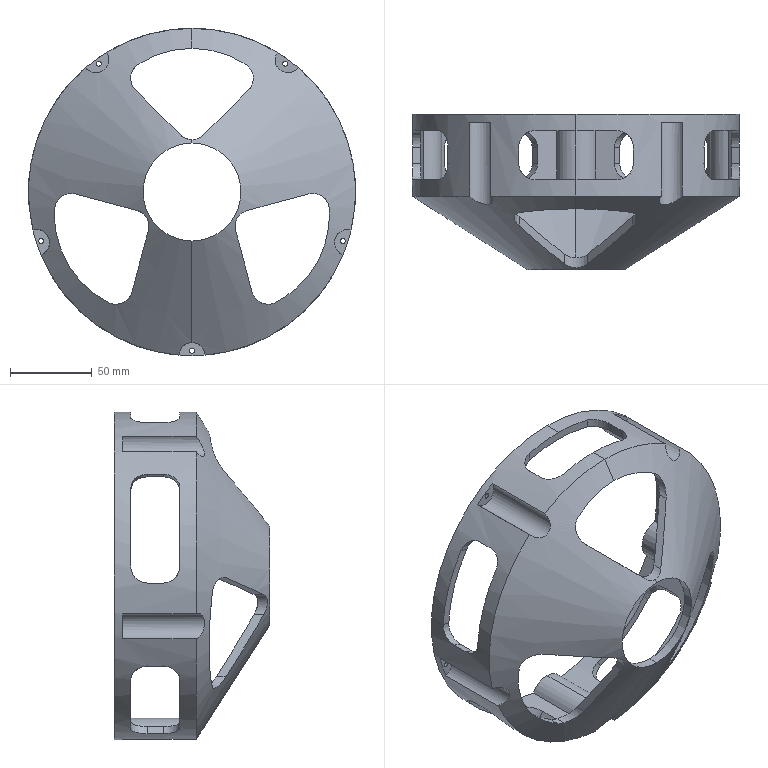Component | SolidWorks | LaserWorkingHeadHood(Lower)-1 | 1 solid | 103 faces | volume 218557 mm3 | cylinder 67 | plane 32 | cone 4 | commonest cylinder face diameters 20 x31 3 x10 16 x8 26 x6 190 x5 120 x3 60 x2 200 x2